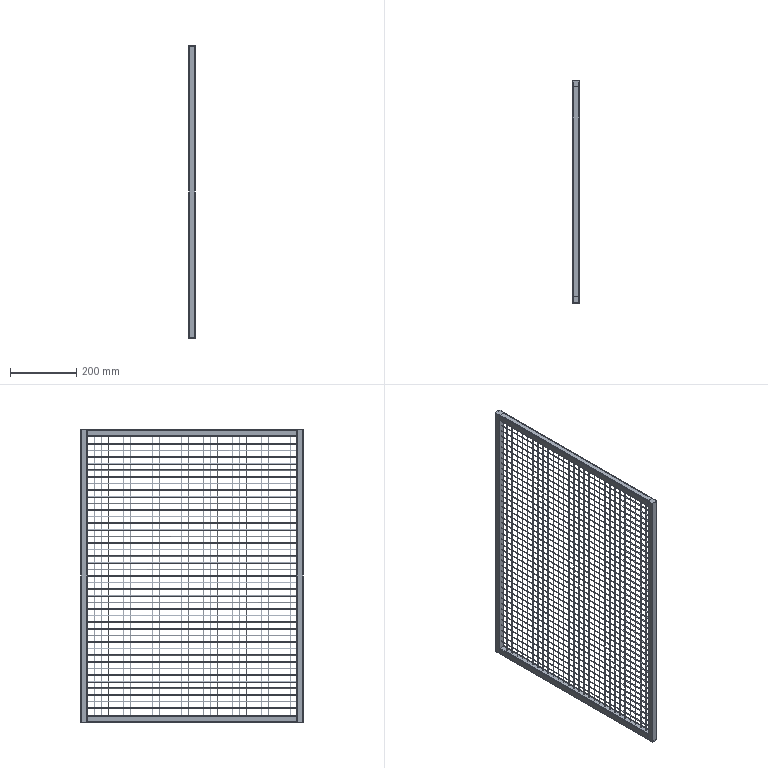Component | NX | FRONT_REAR_BAFFLE | 77 solids | 319 faces | volume 381918 mm3 | plane 202 | cylinder 117 | commonest cylinder face diameters 2 x101 4 x16